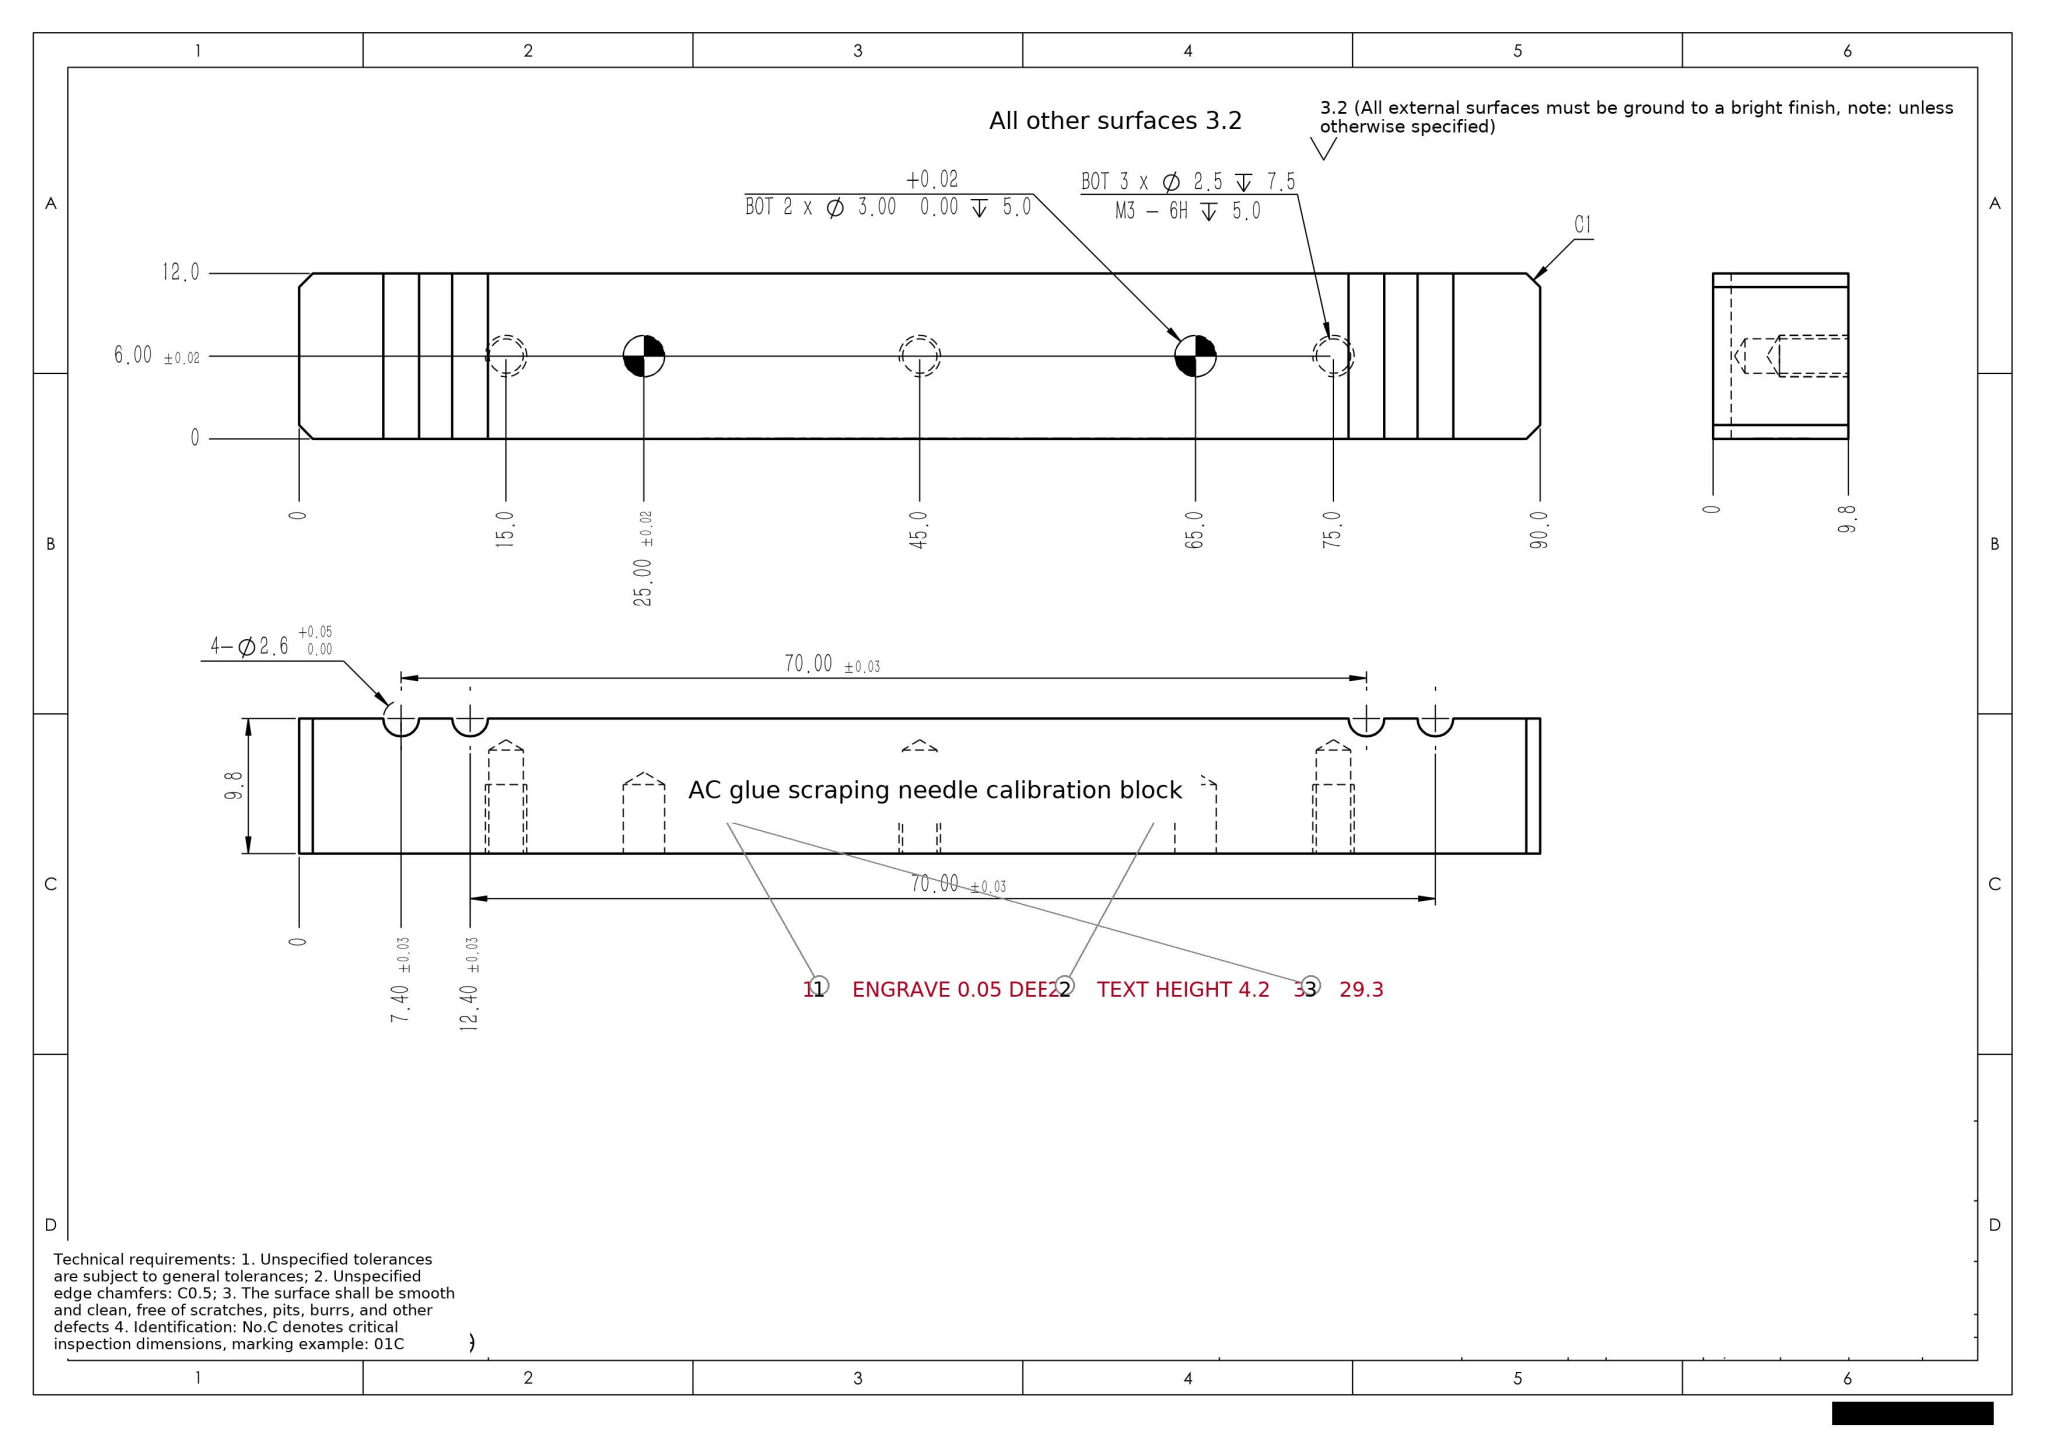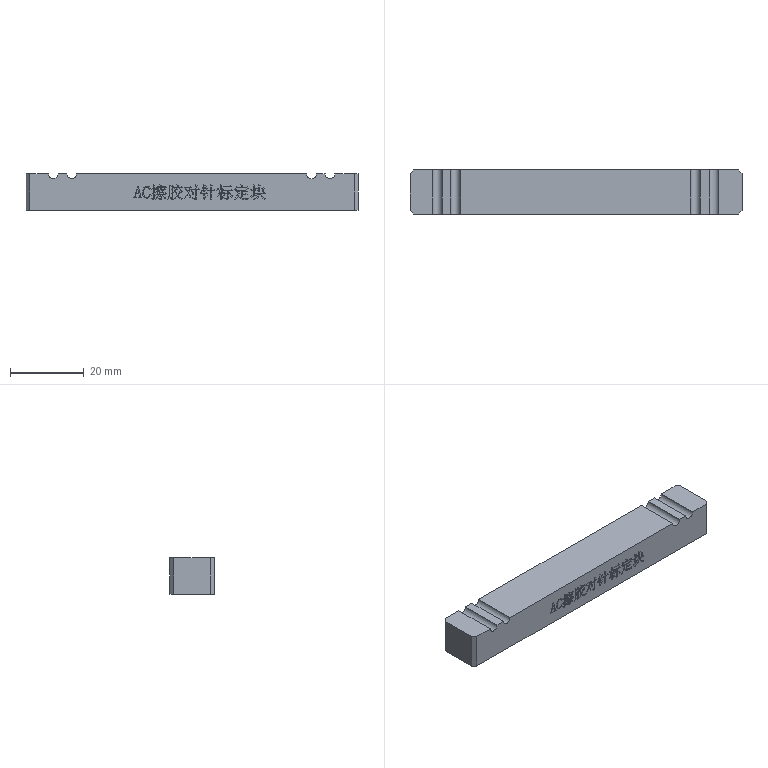Part | SolidWorks | mm | 1 solid | 481 faces | box 90 x 12 x 9.8 mm | volume 10247 mm3 | plane 333 | spline 124 | cylinder 14 | cone 10 | commonest cylinder face diameters 2.5 x6 3 x4 2.6 x4